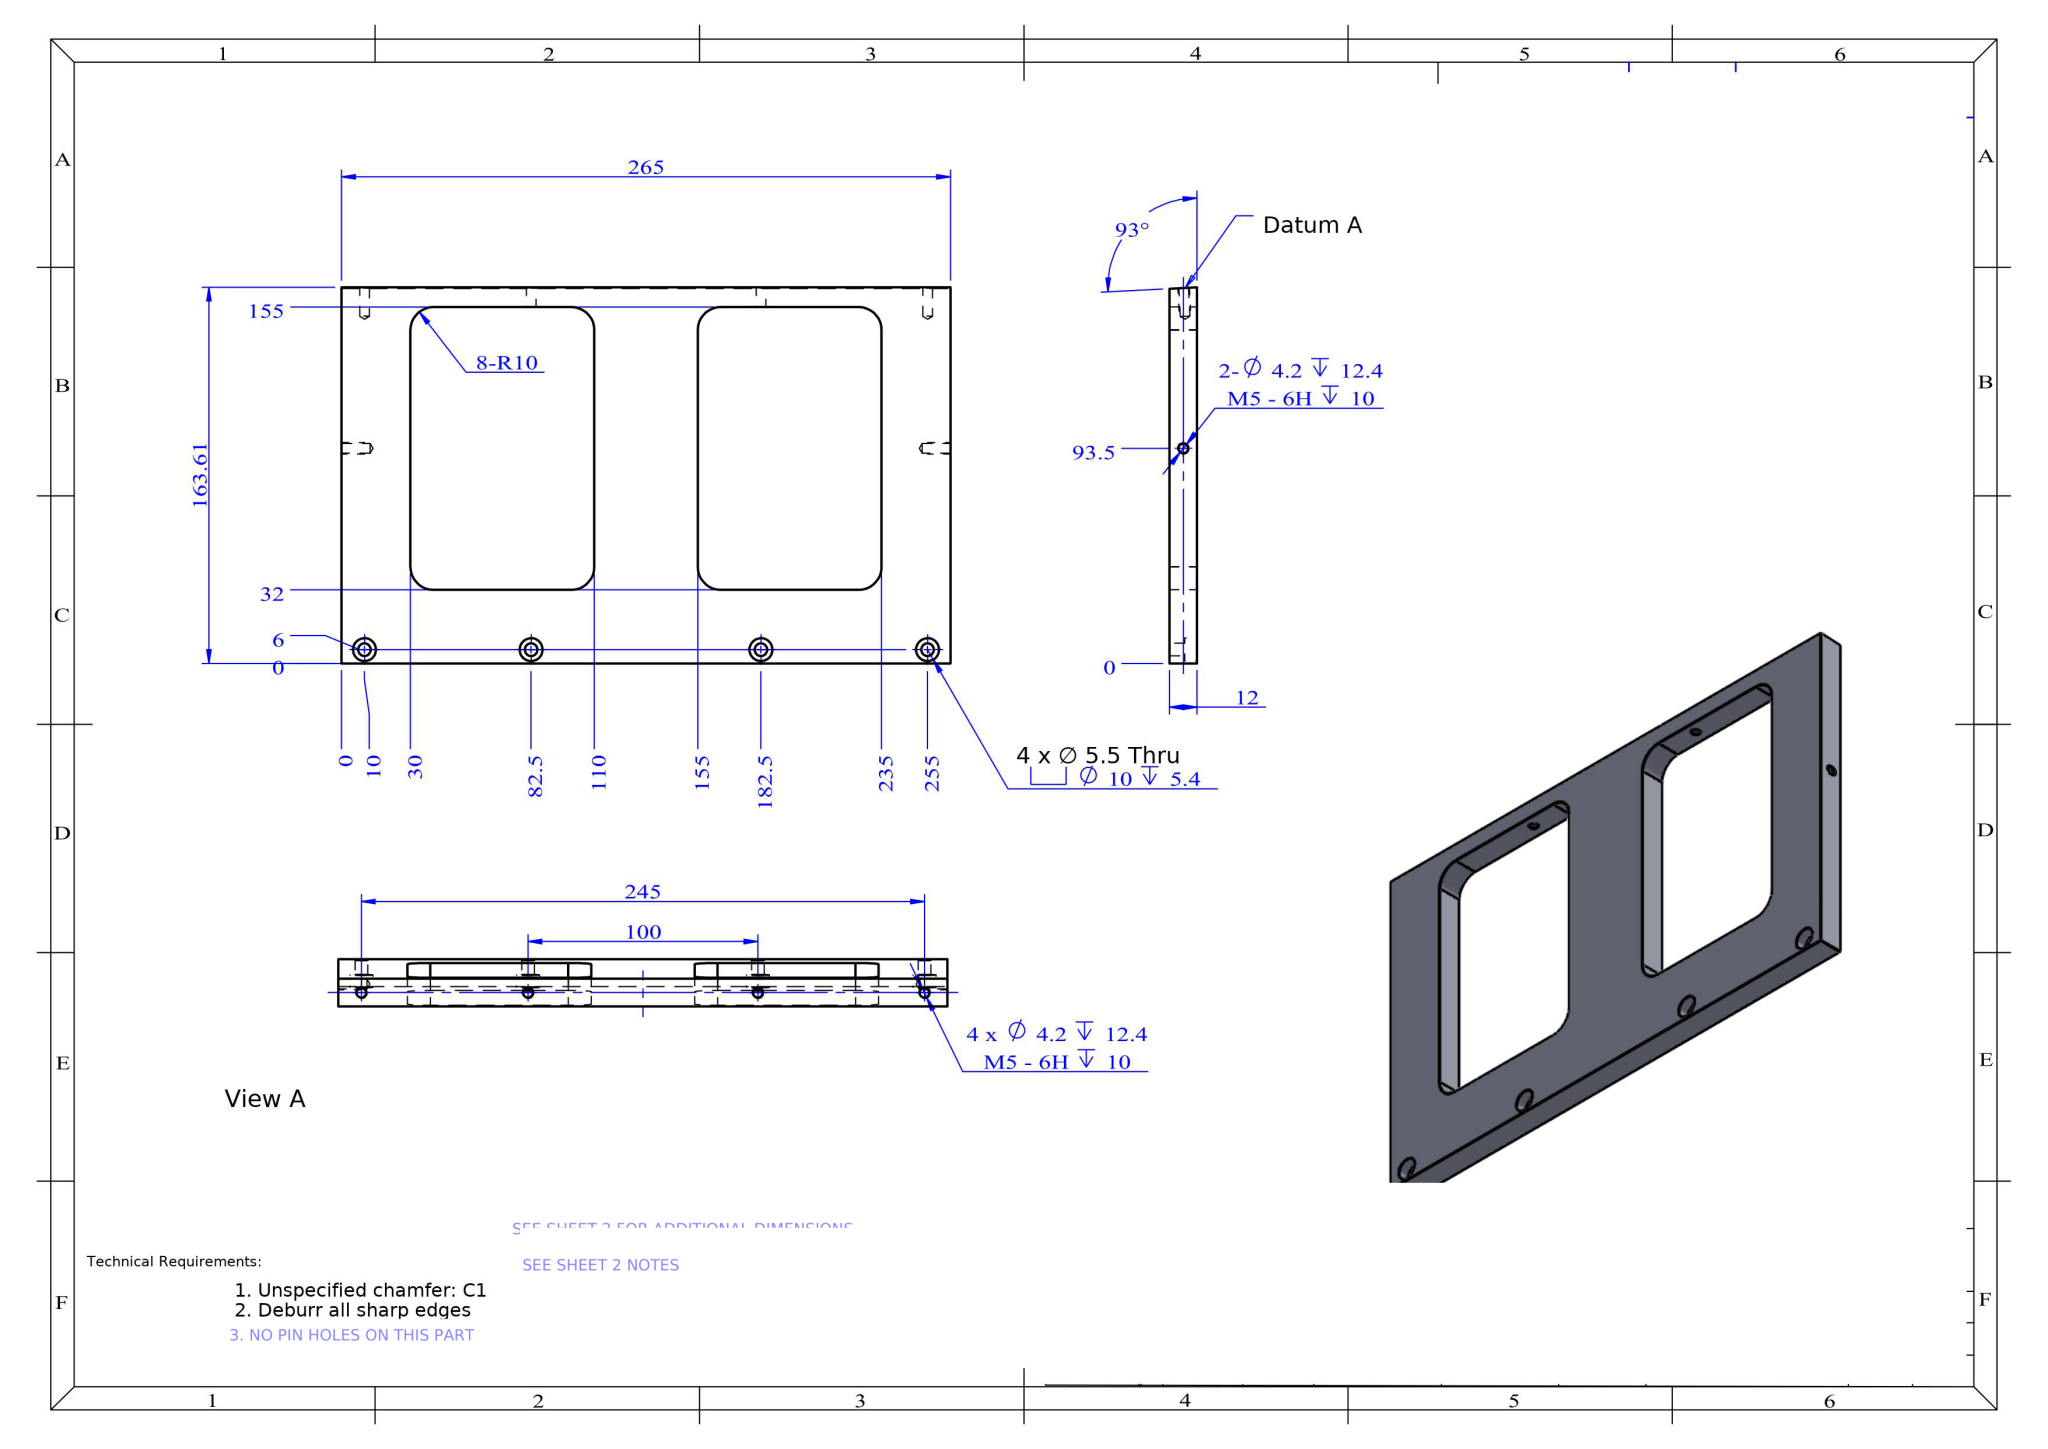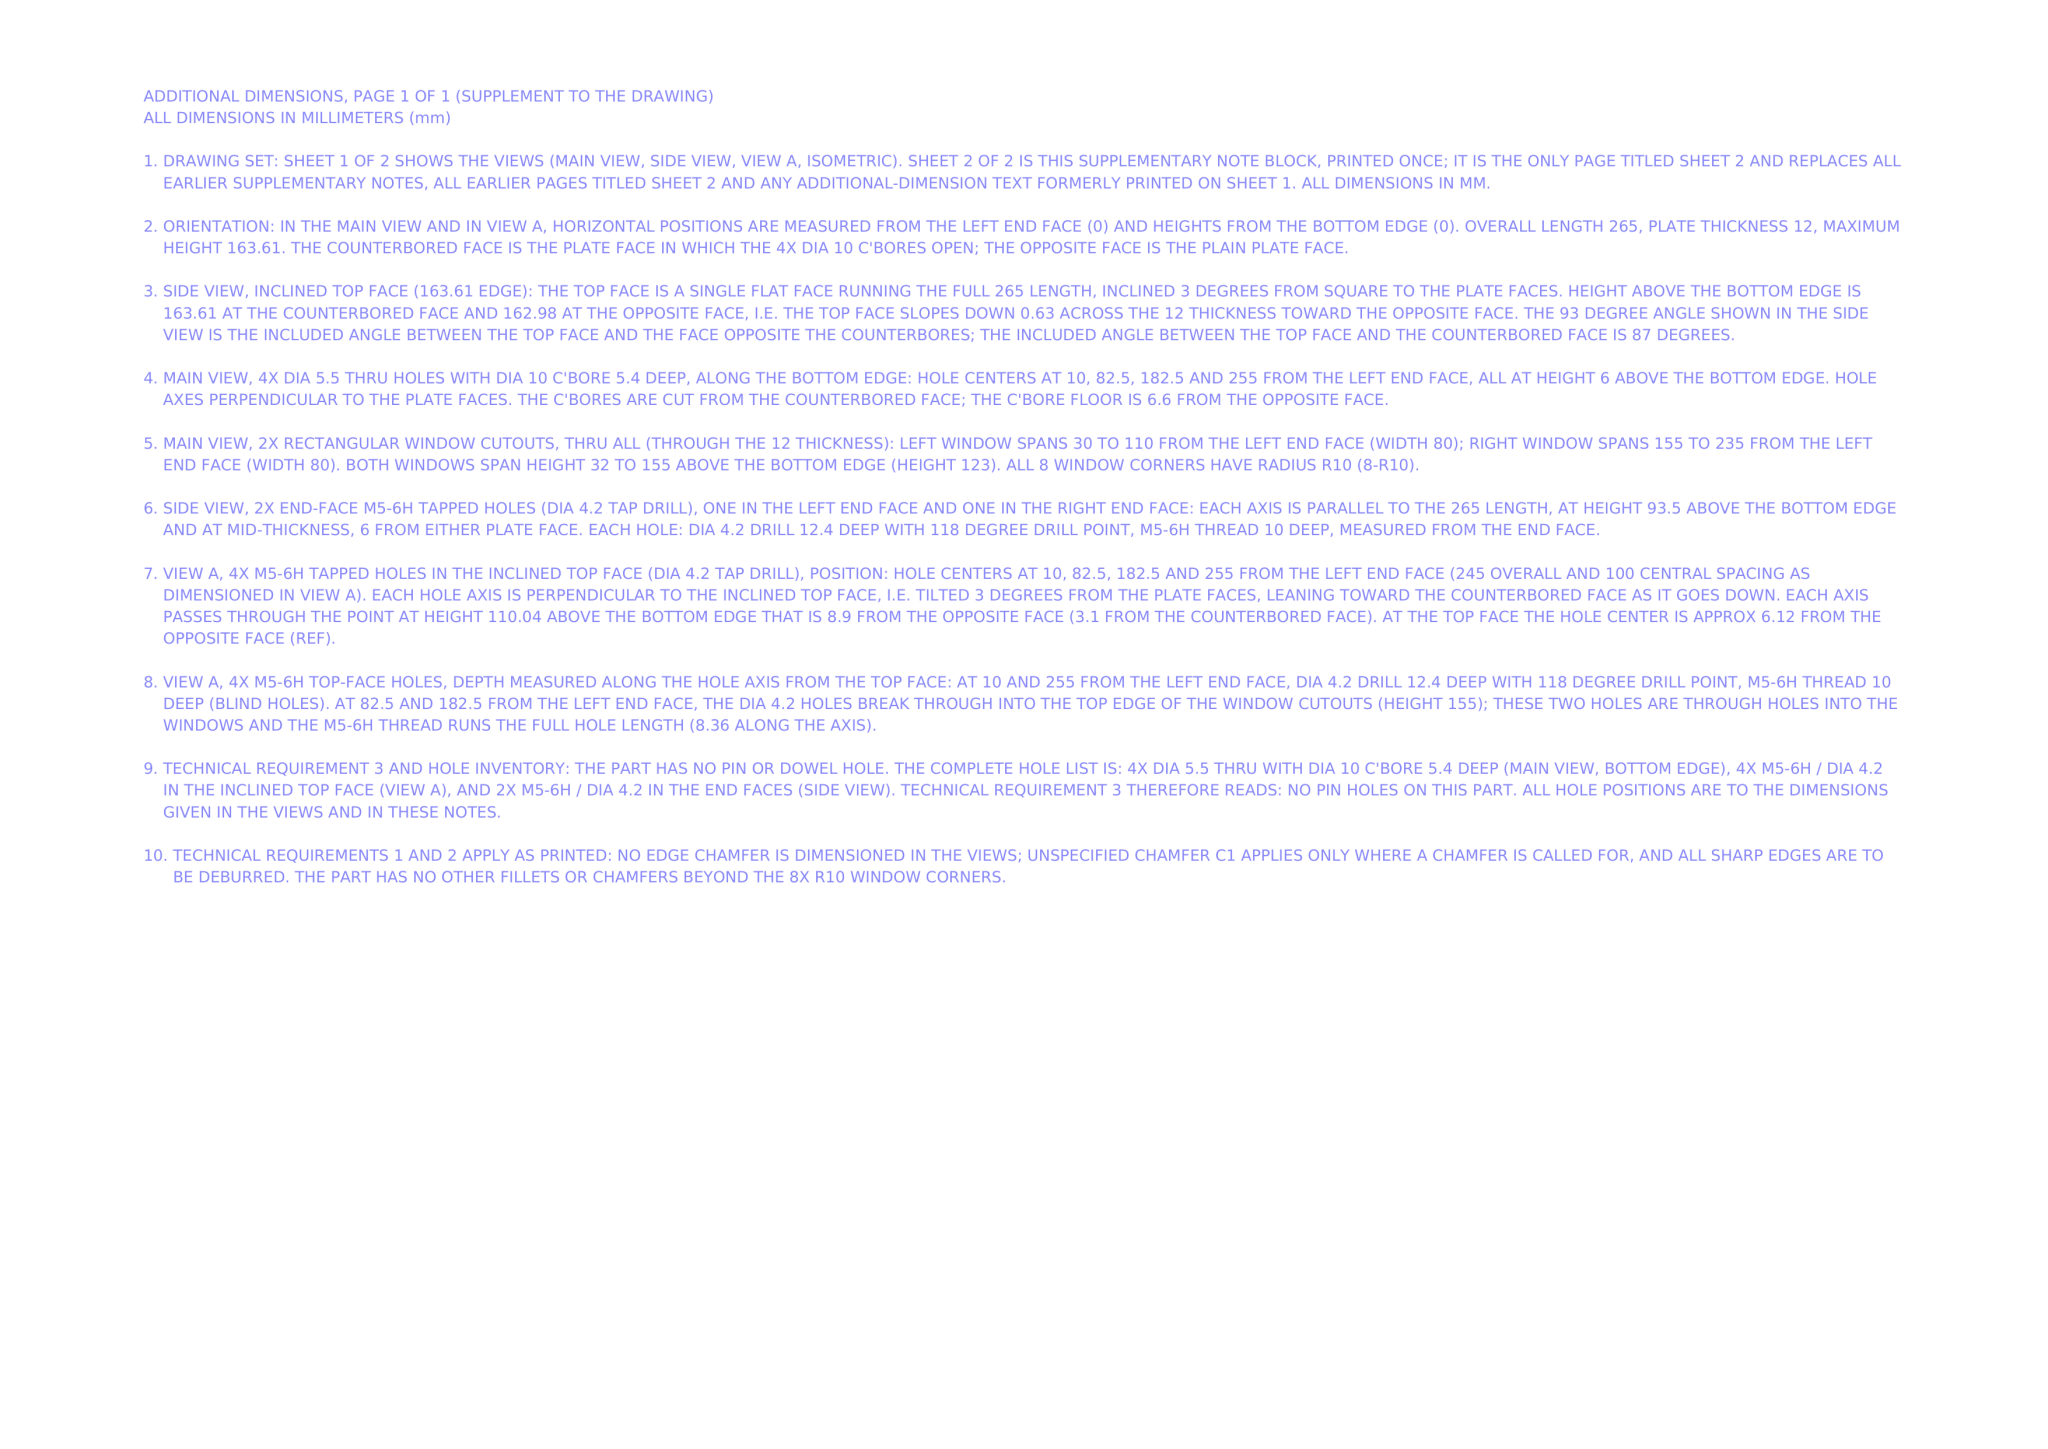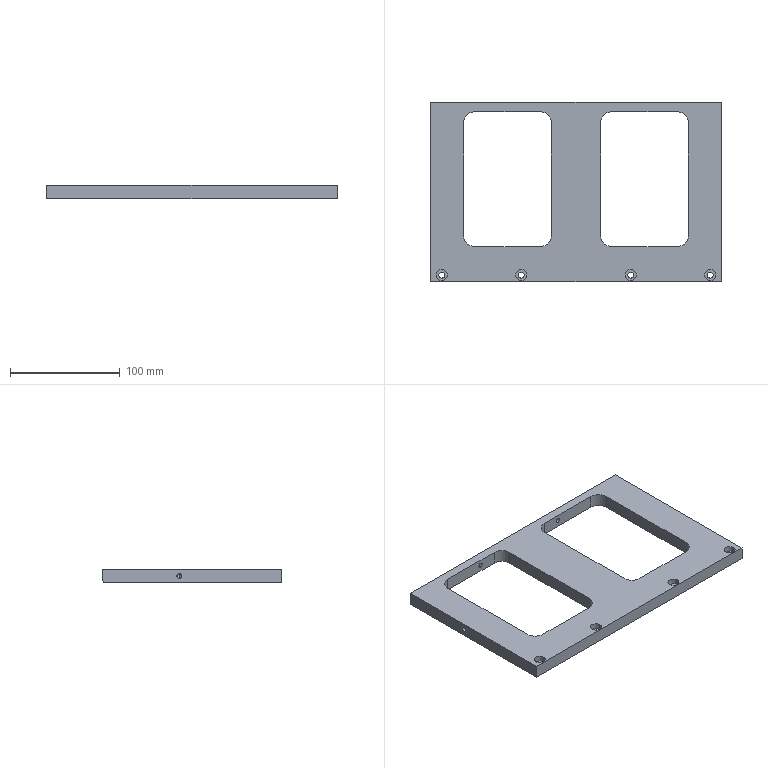Part | NX | mm | 1 solid | 62 faces | box 265 x 163.61 x 12 mm | volume 281923 mm3 | cylinder 36 | plane 18 | cone 8 | commonest cylinder face diameters 4.2 x12 10 x8 5.5 x8 20 x8